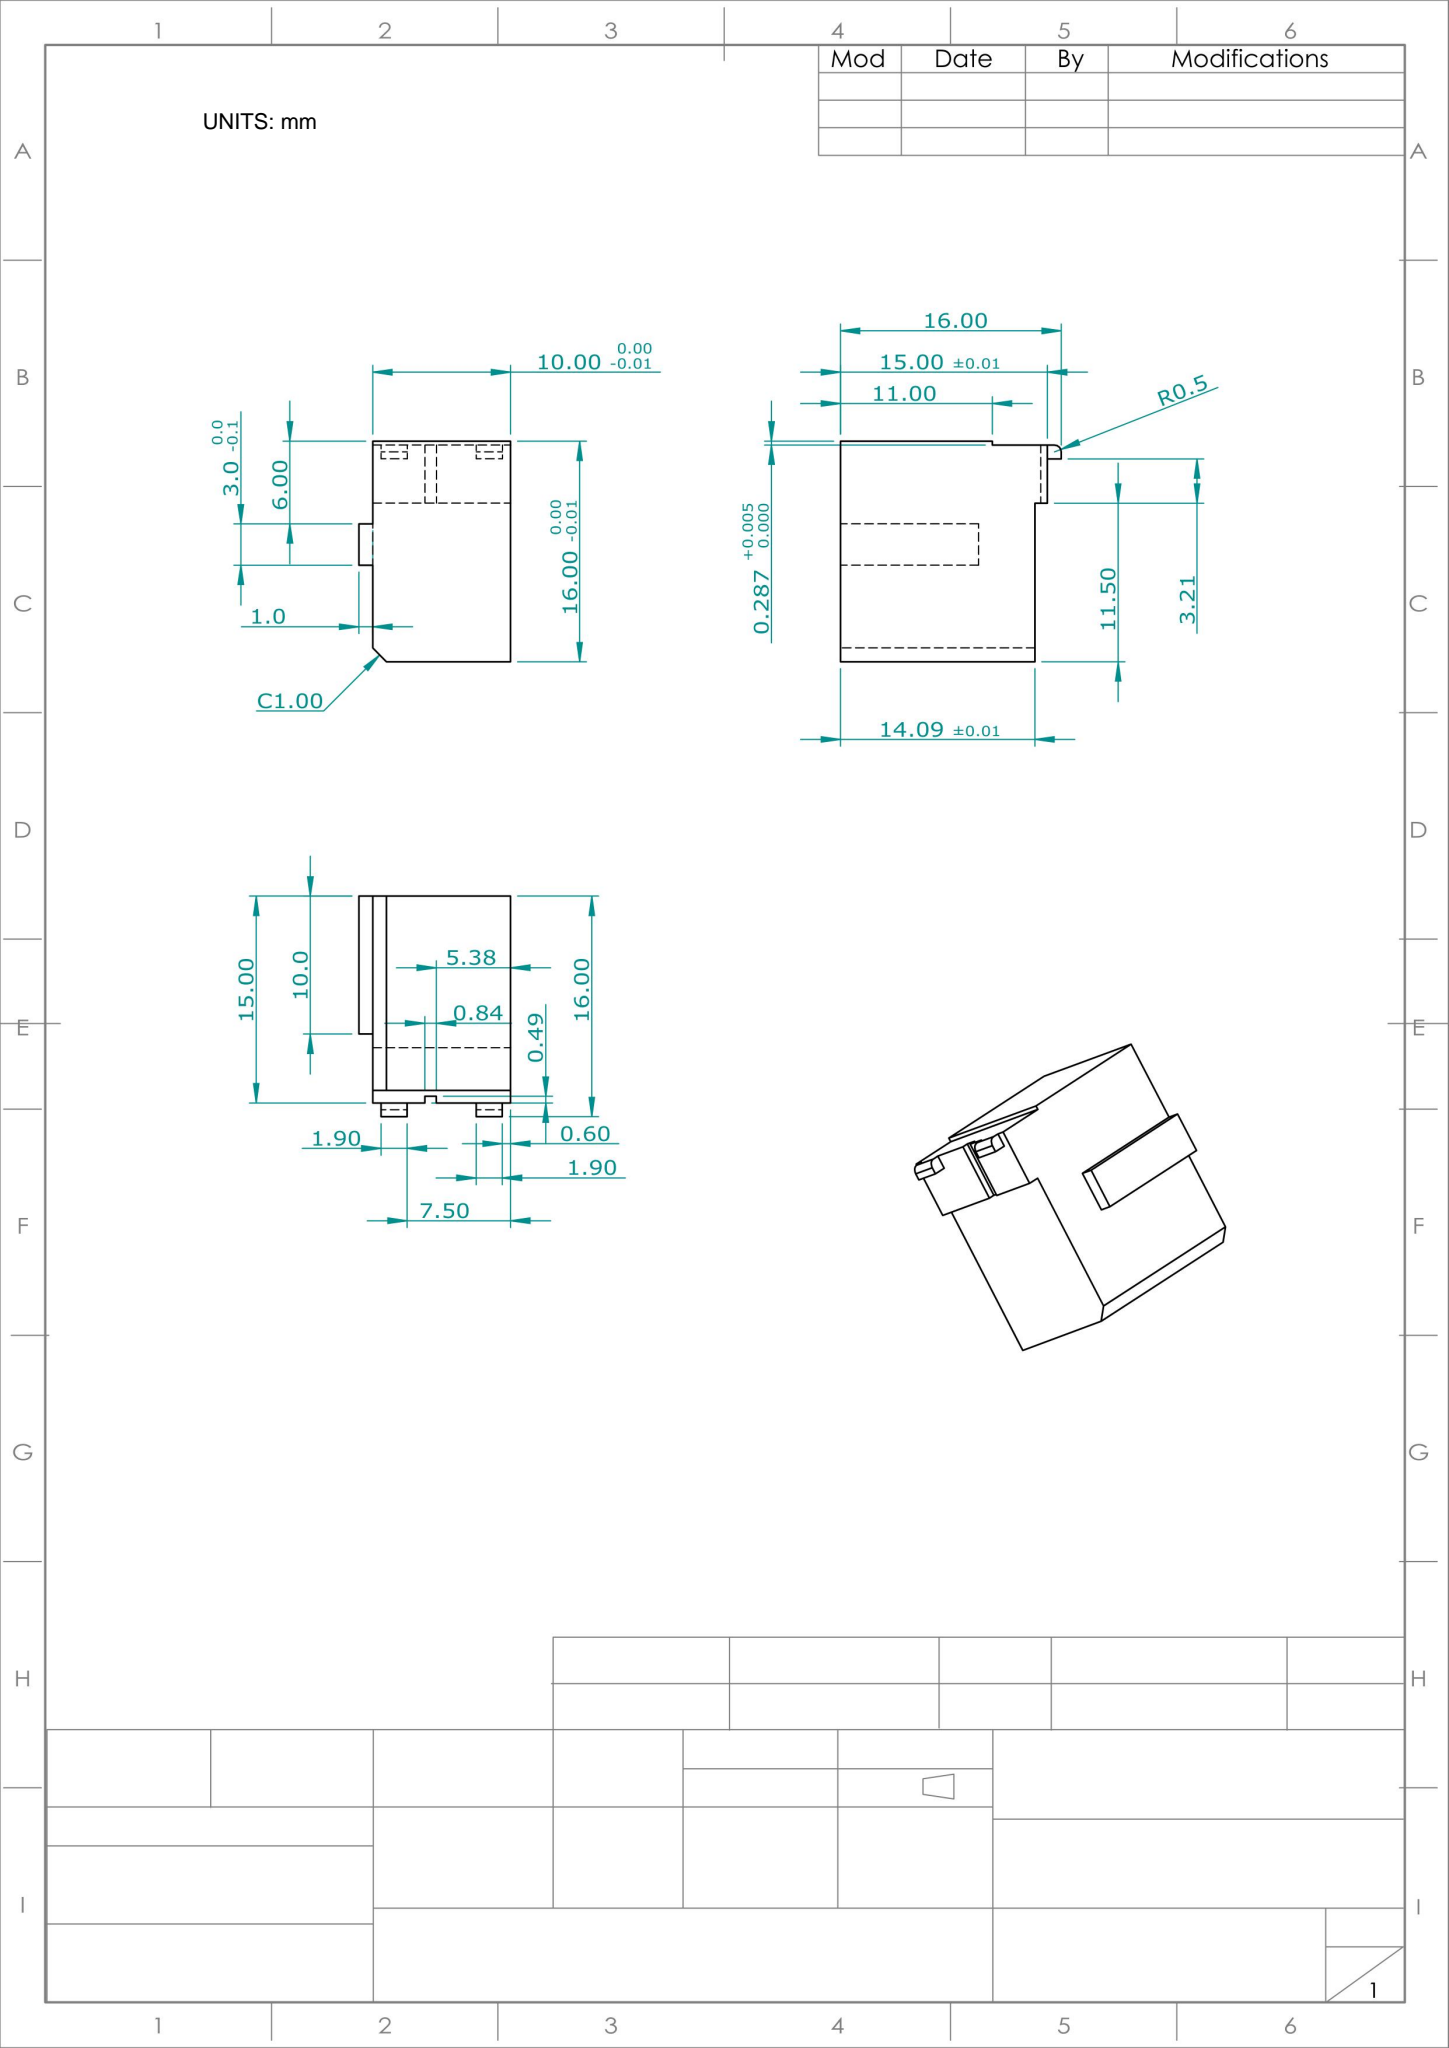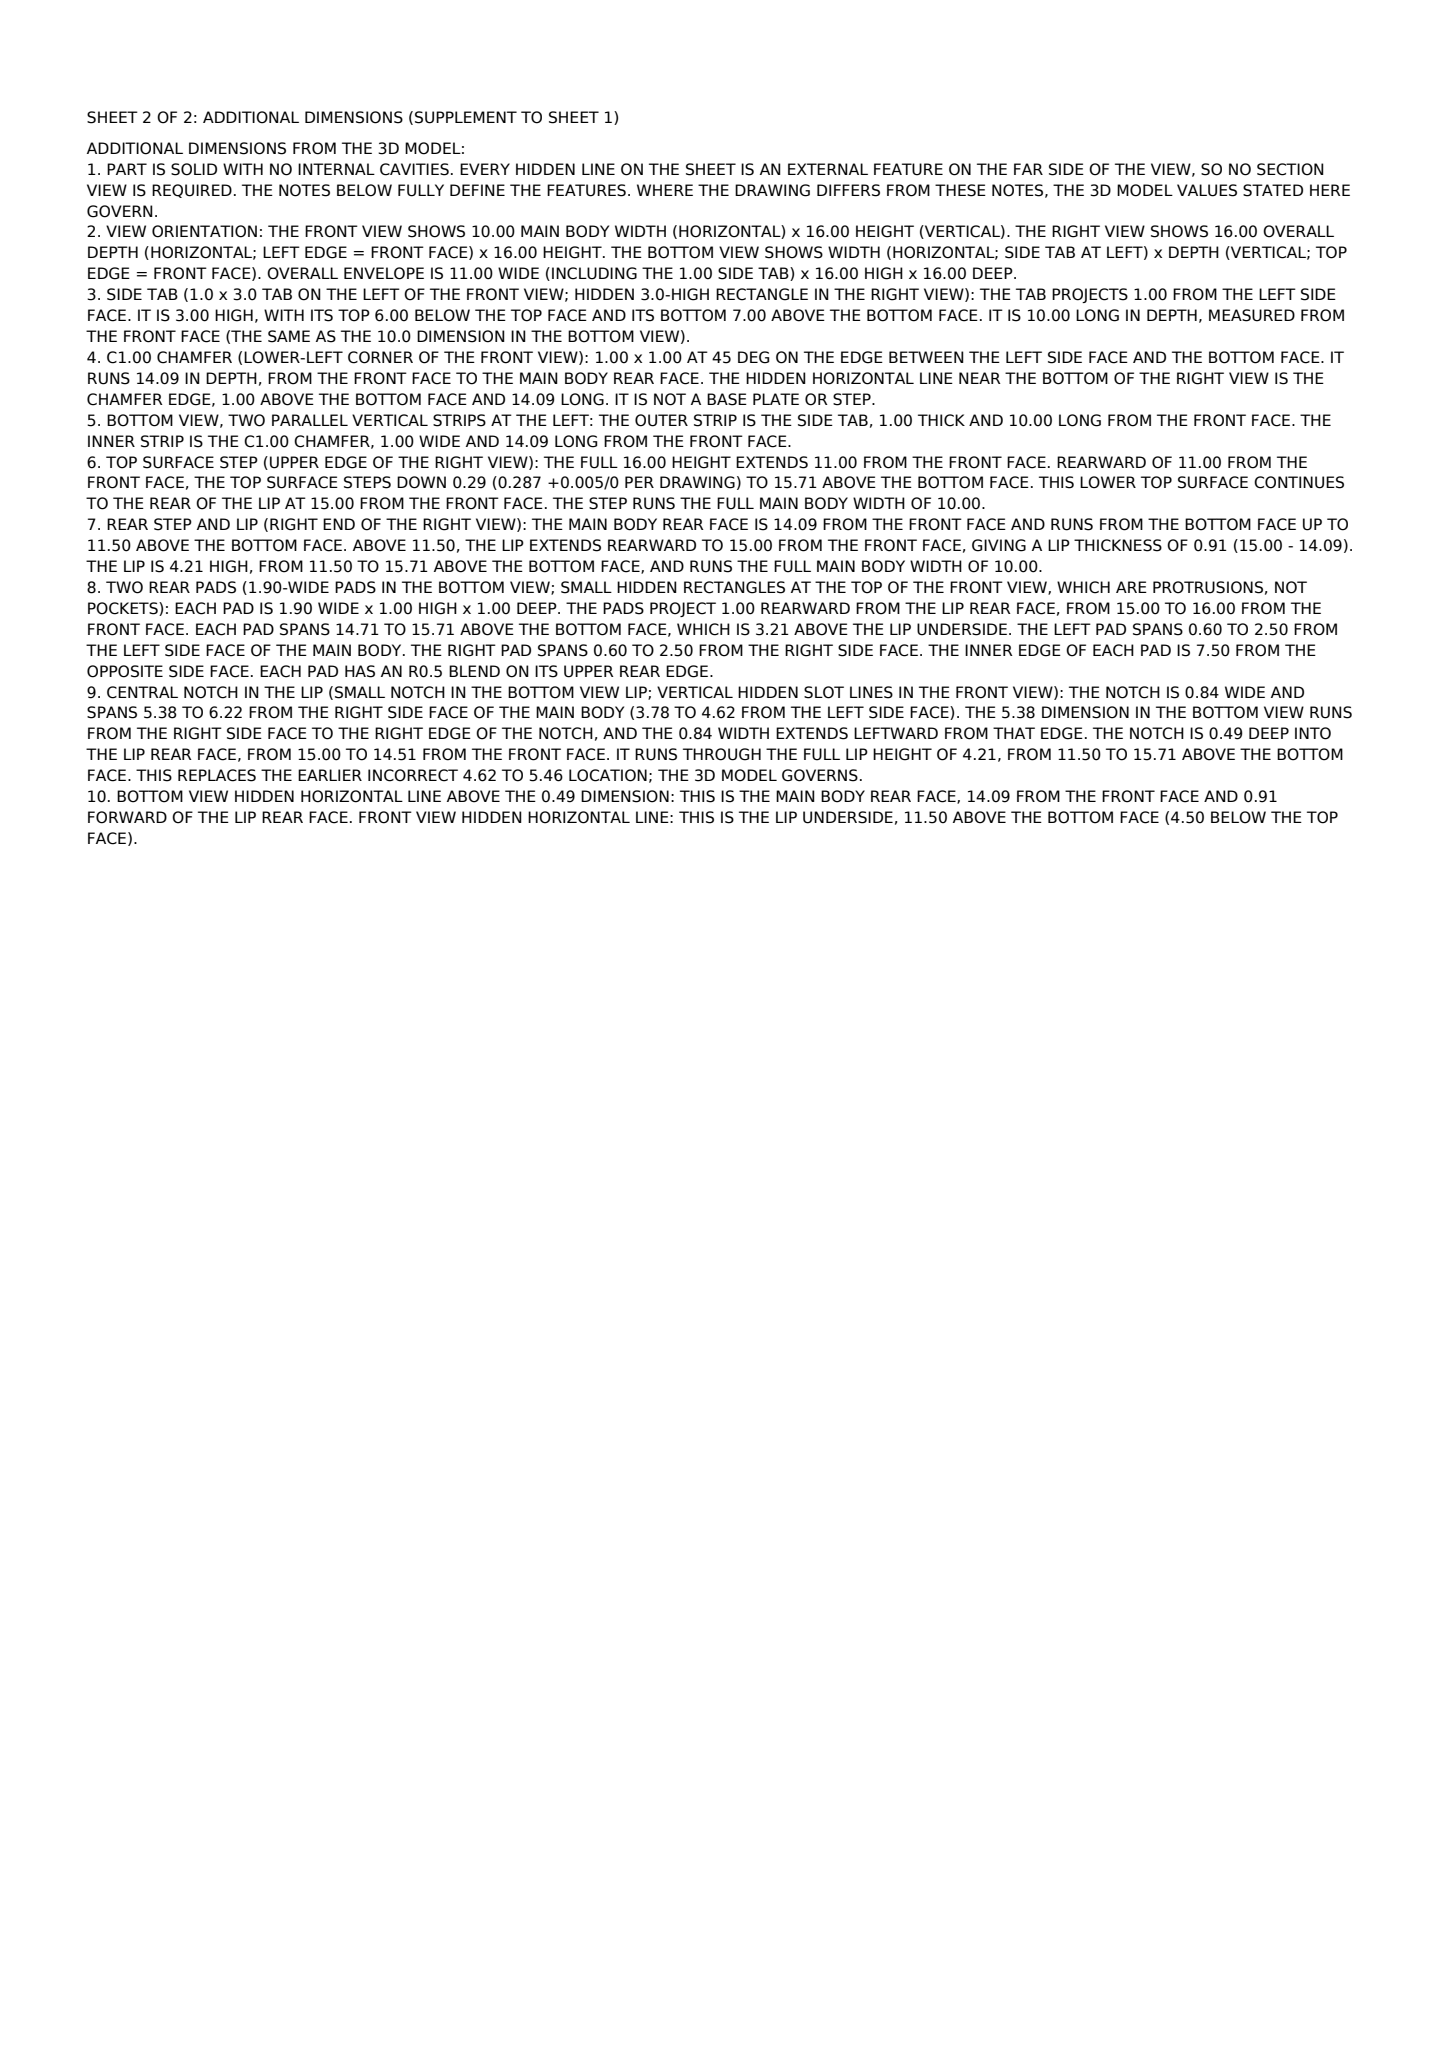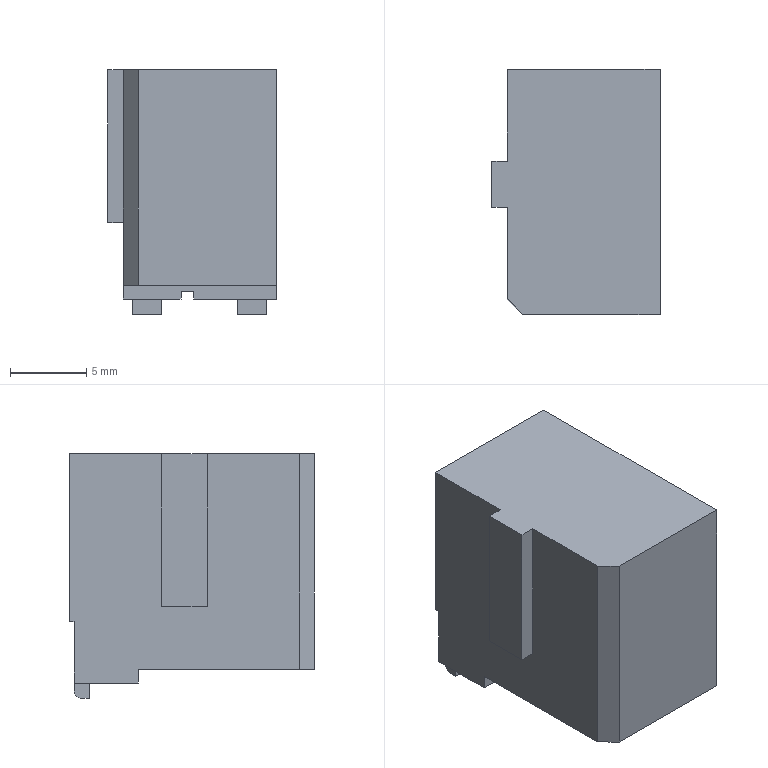Part | NX | mm | 1 solid | 29 faces | box 11 x 16 x 16 mm | volume 2309 mm3 | plane 27 | cylinder 2 | commonest cylinder face diameters 1 x2